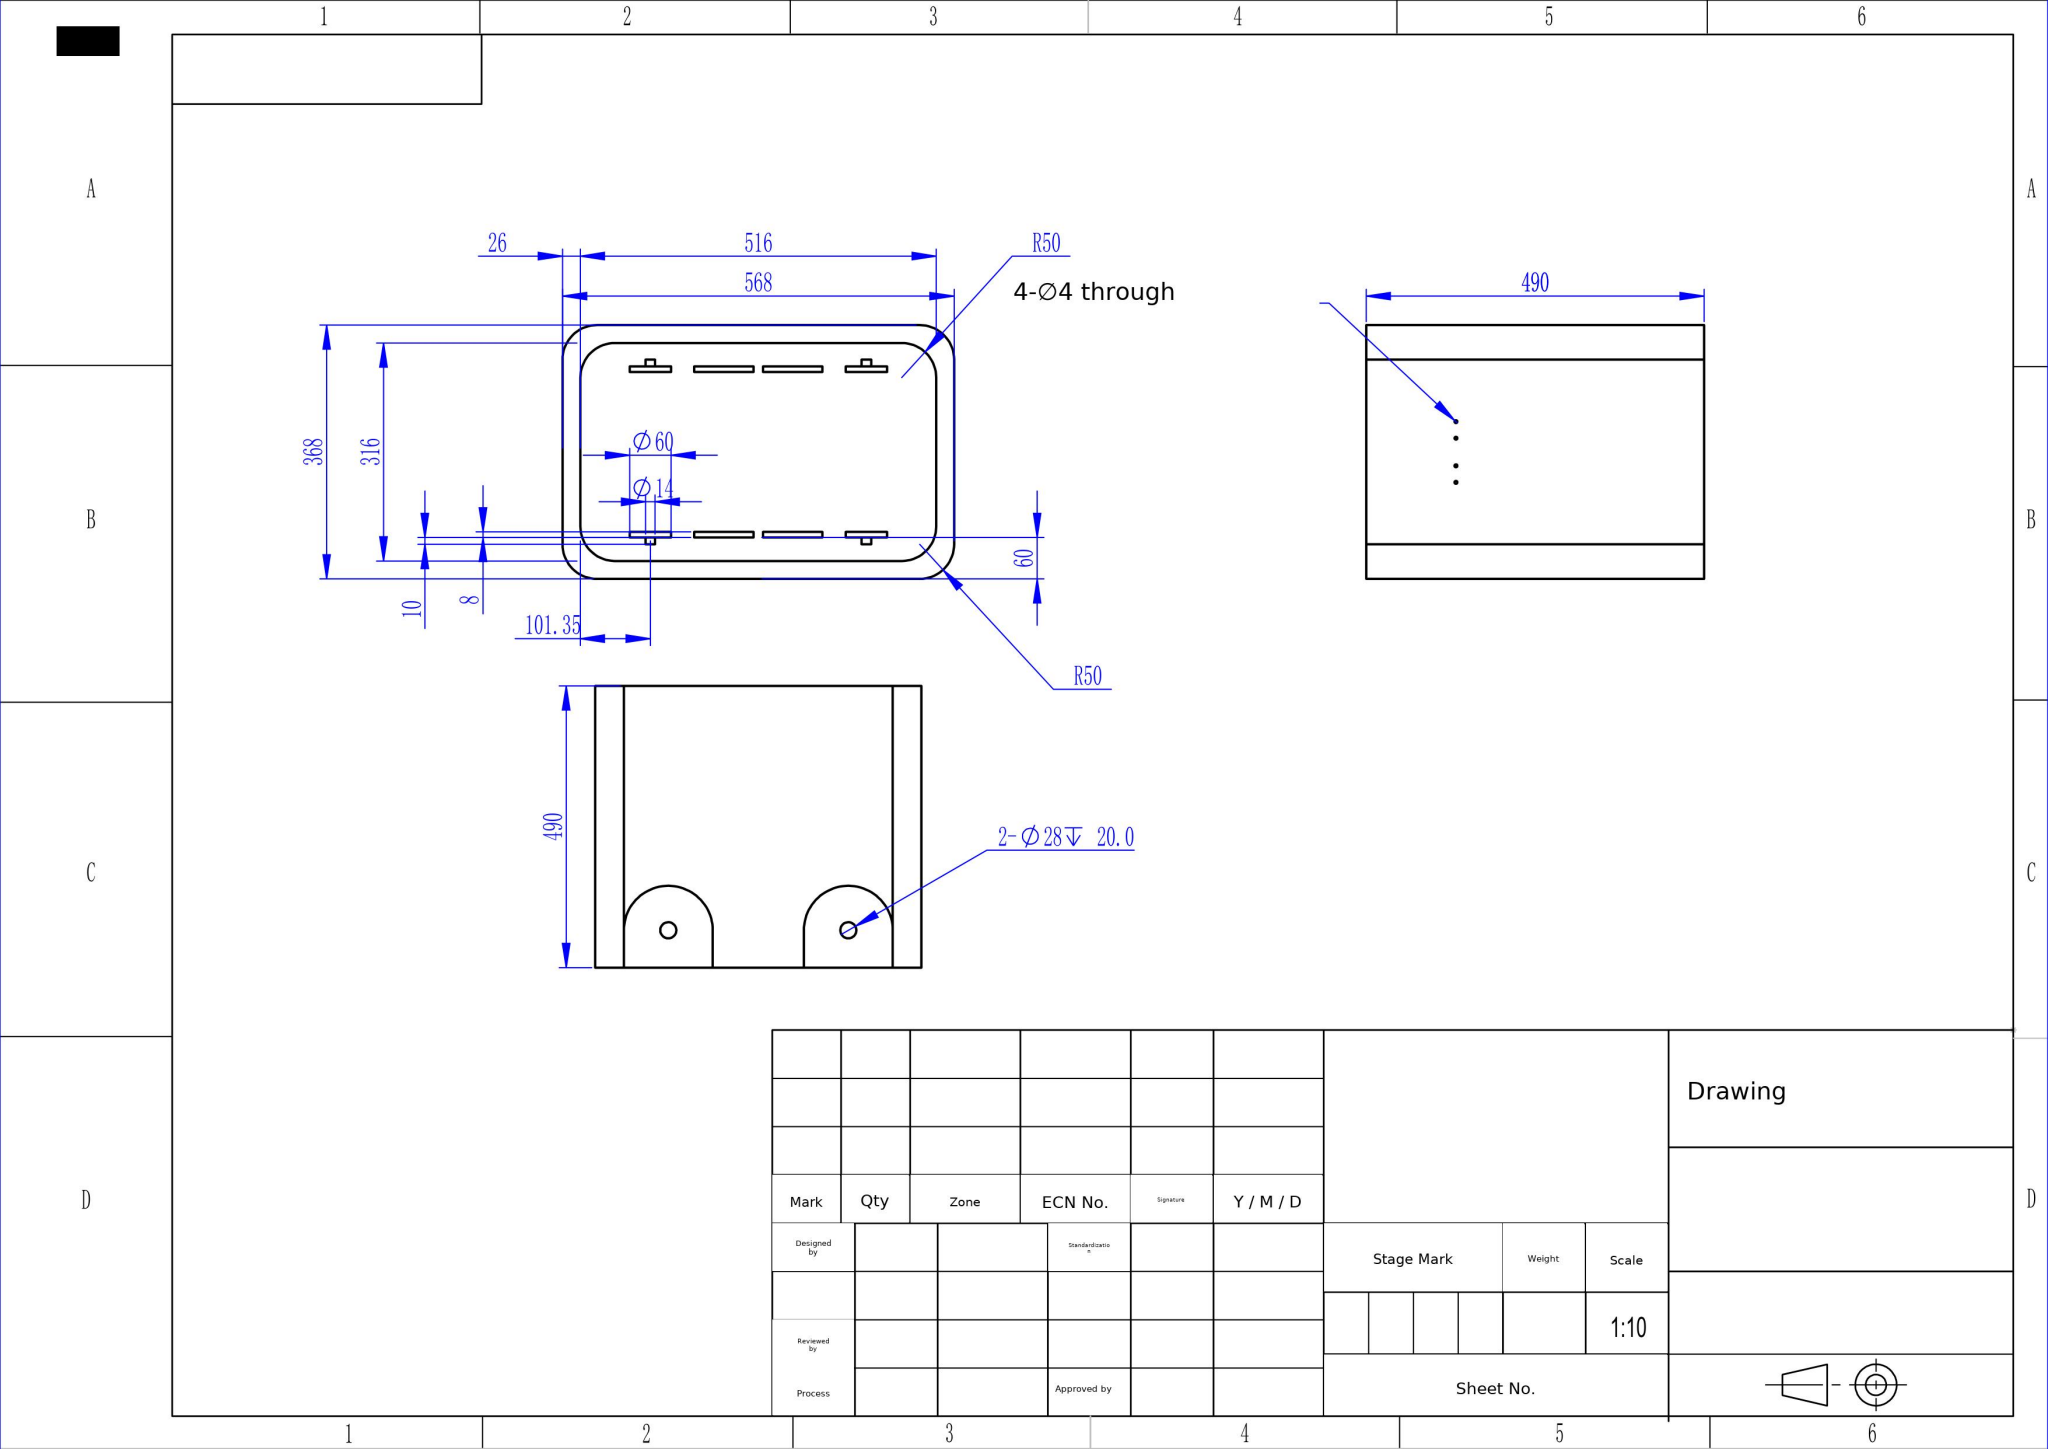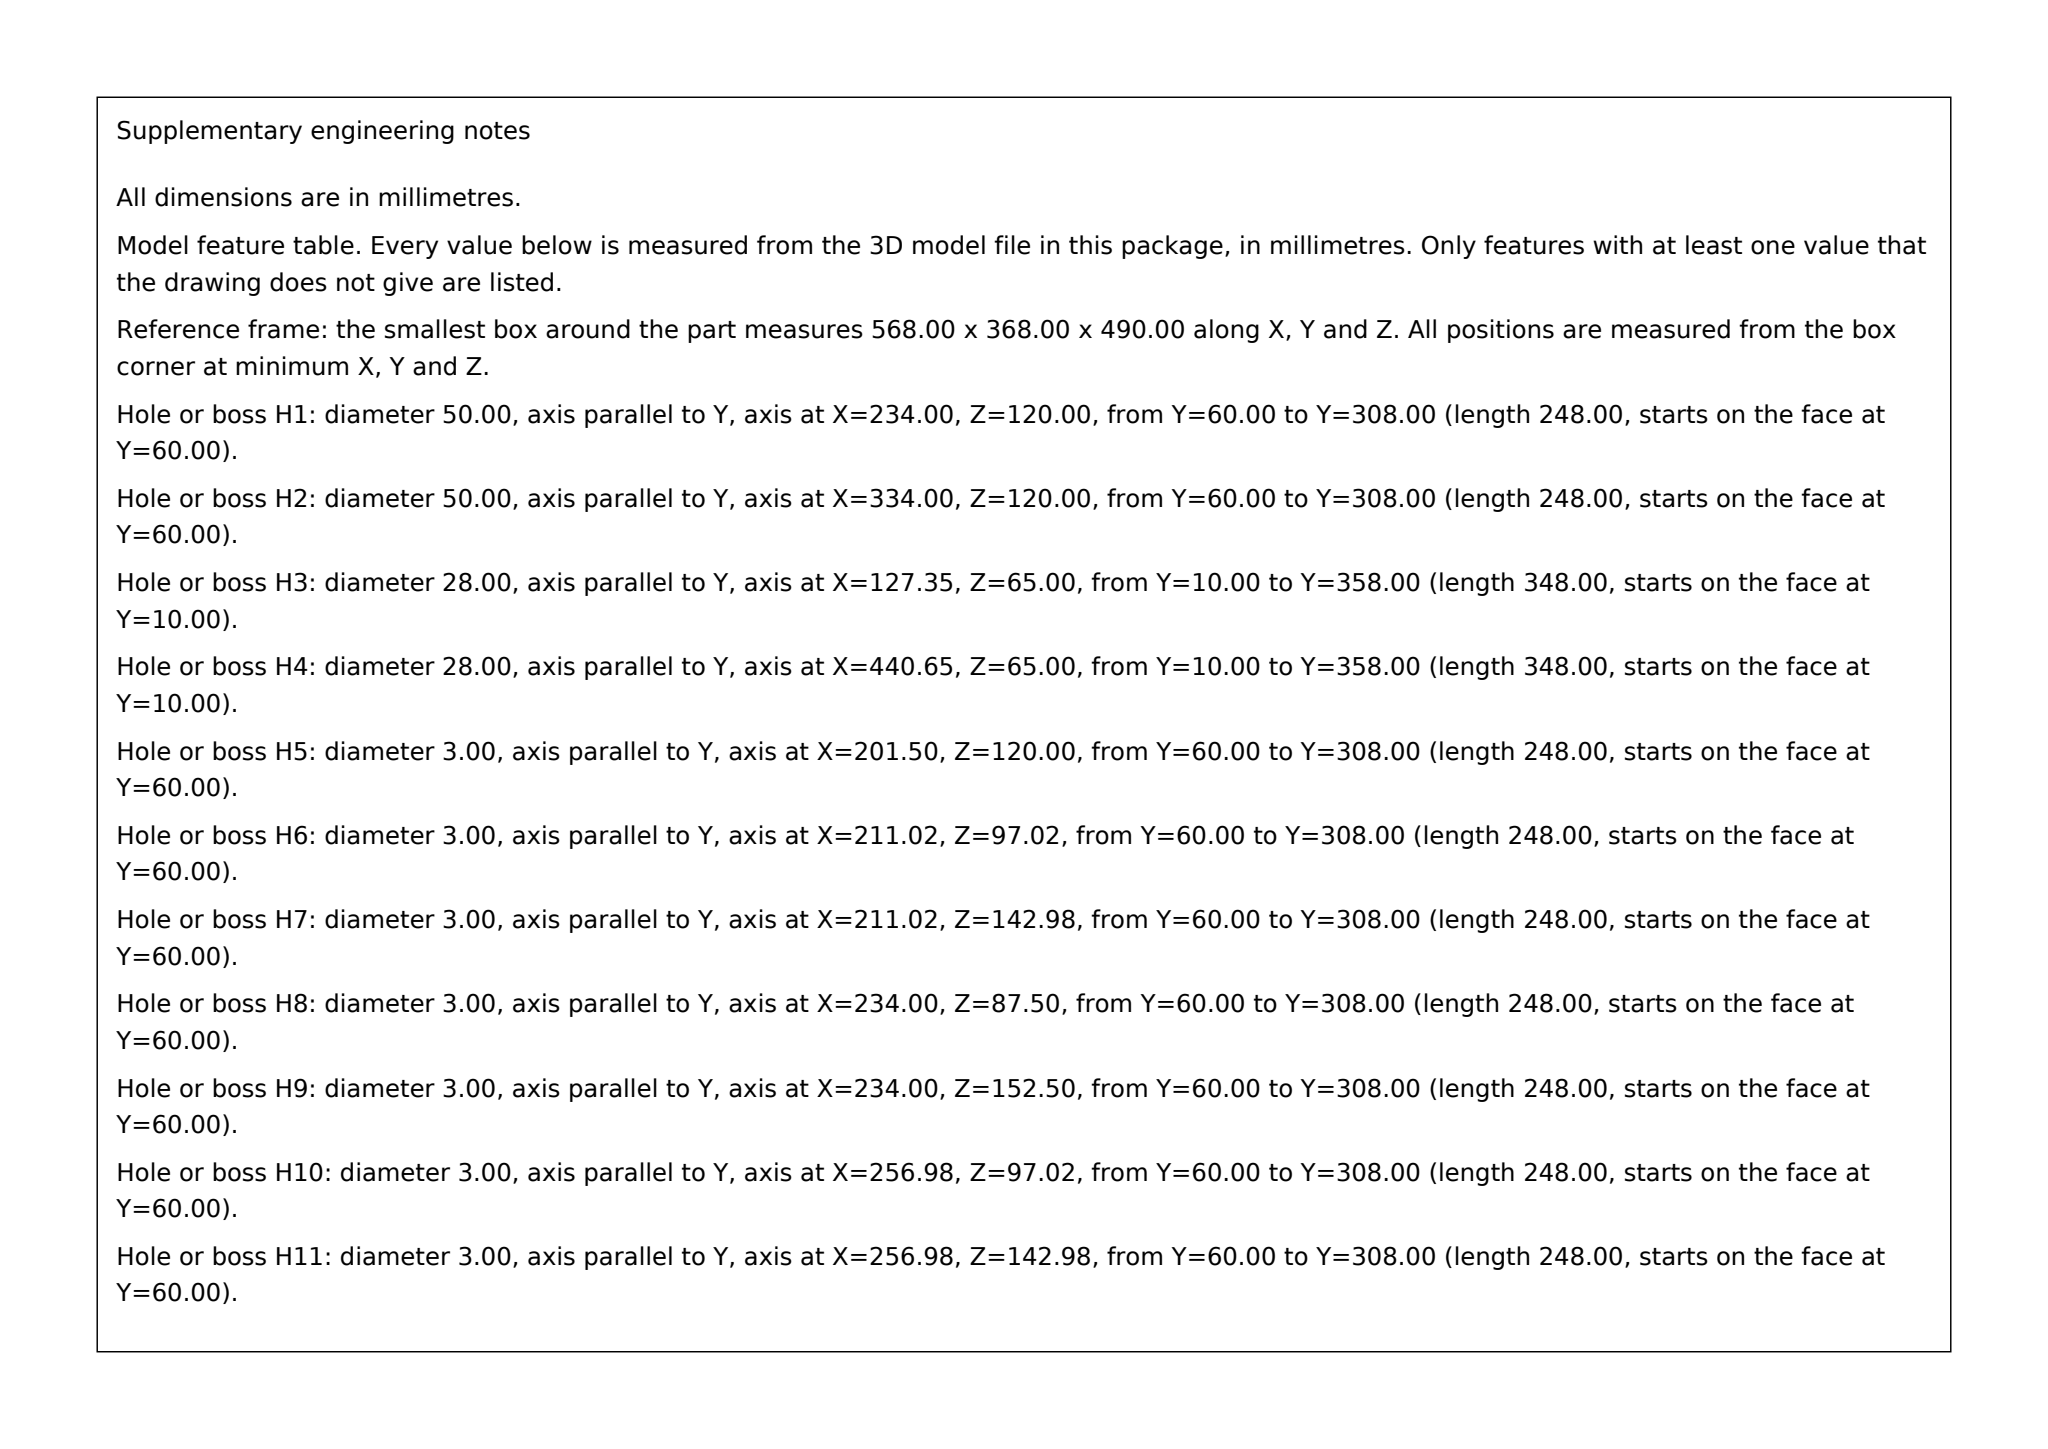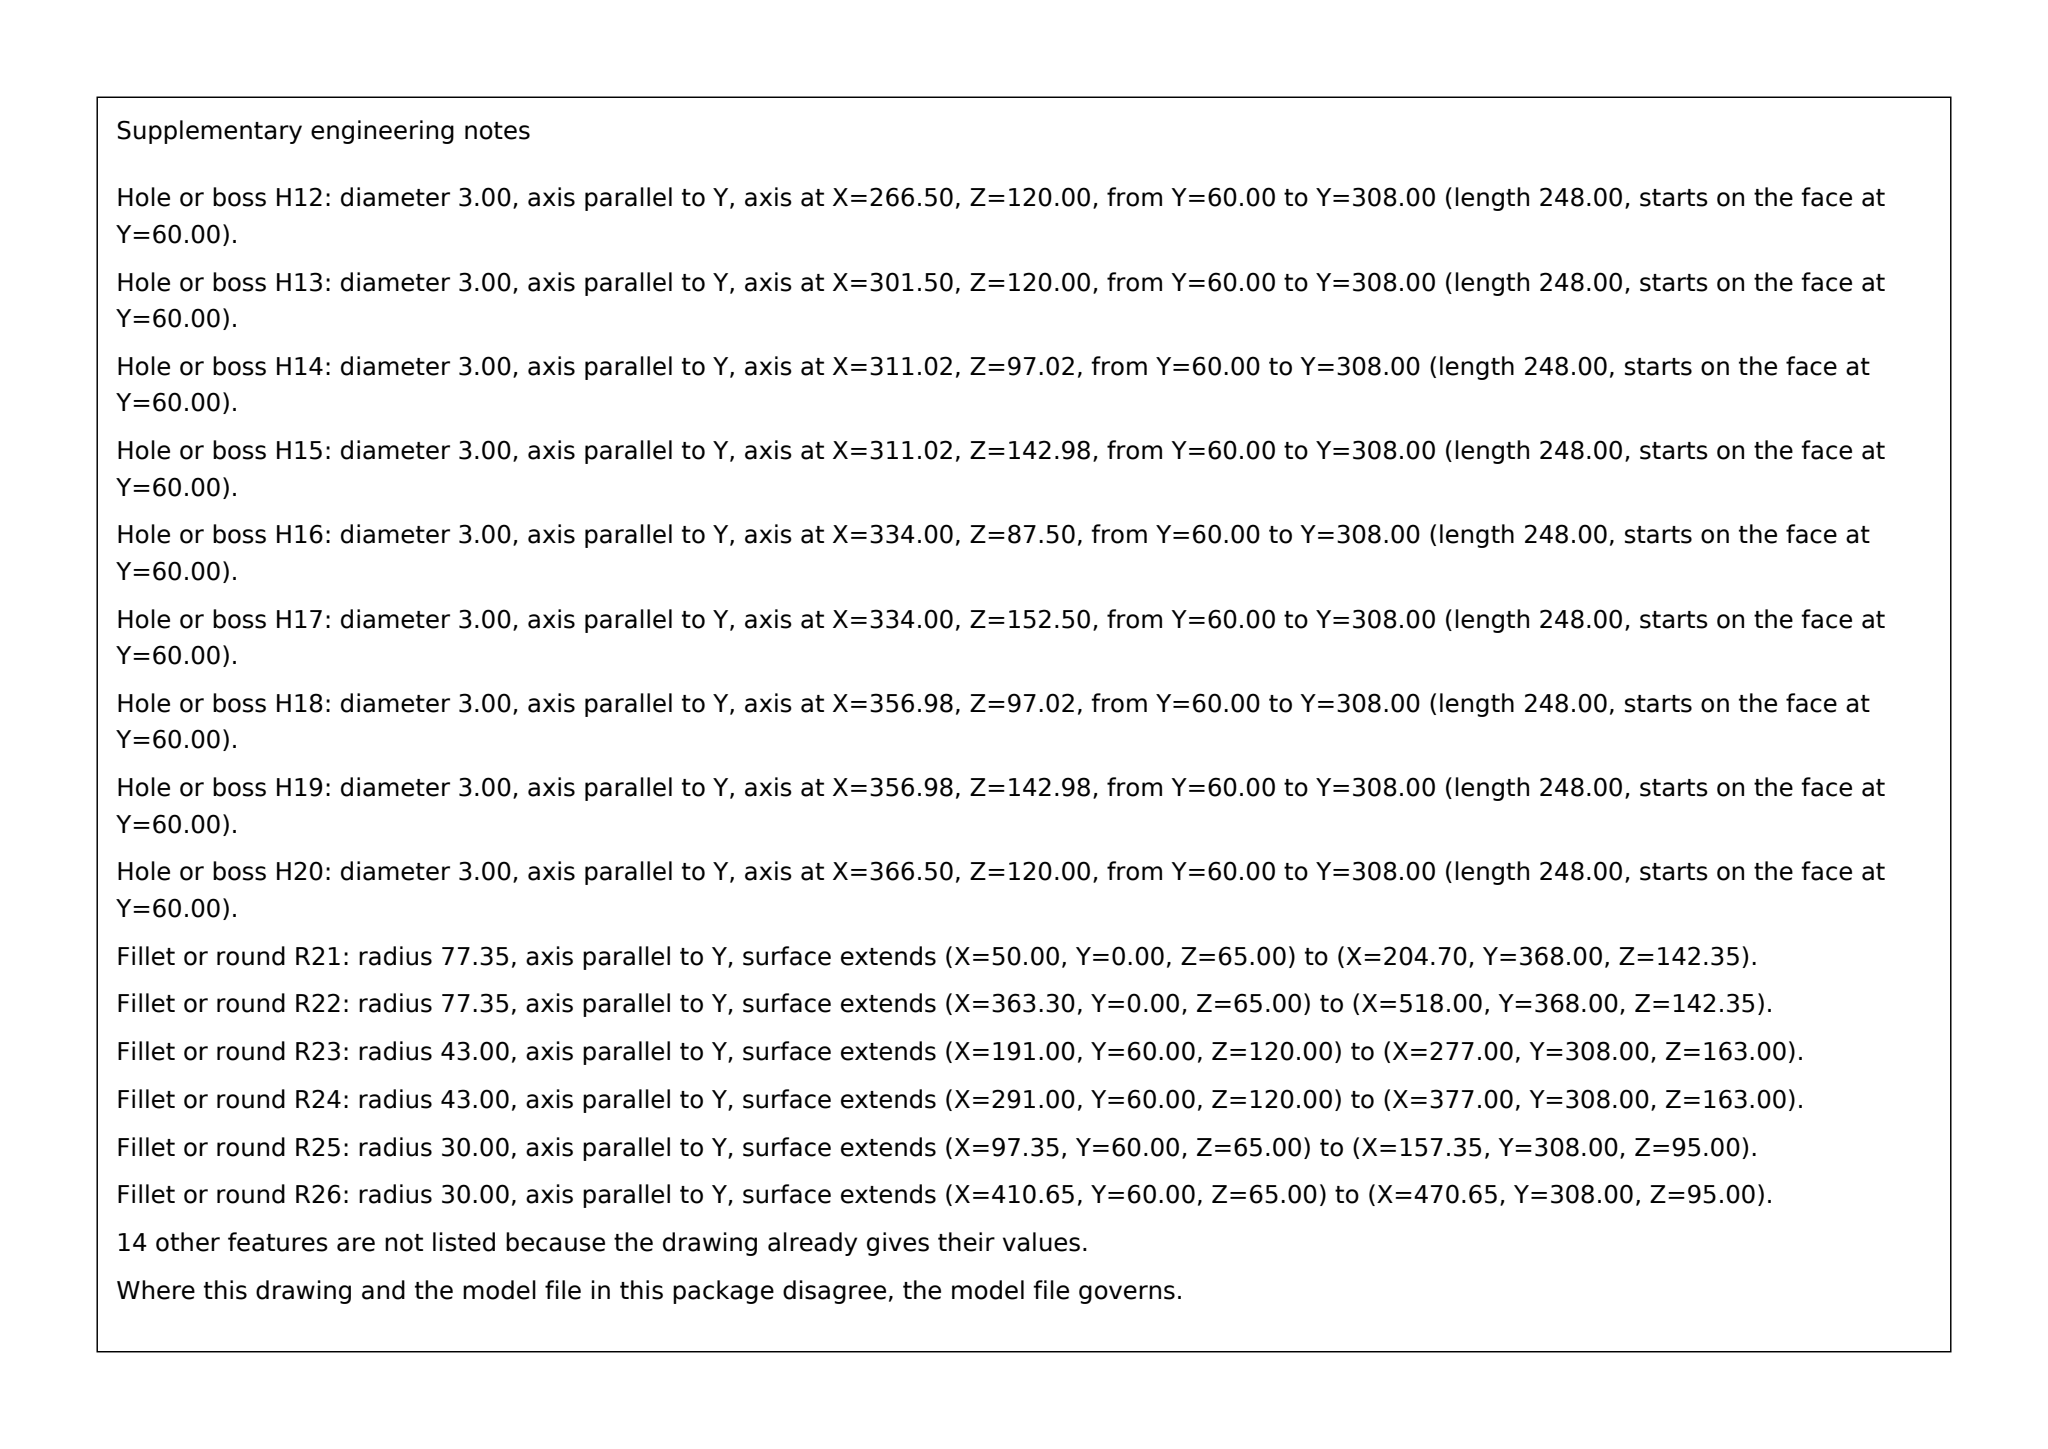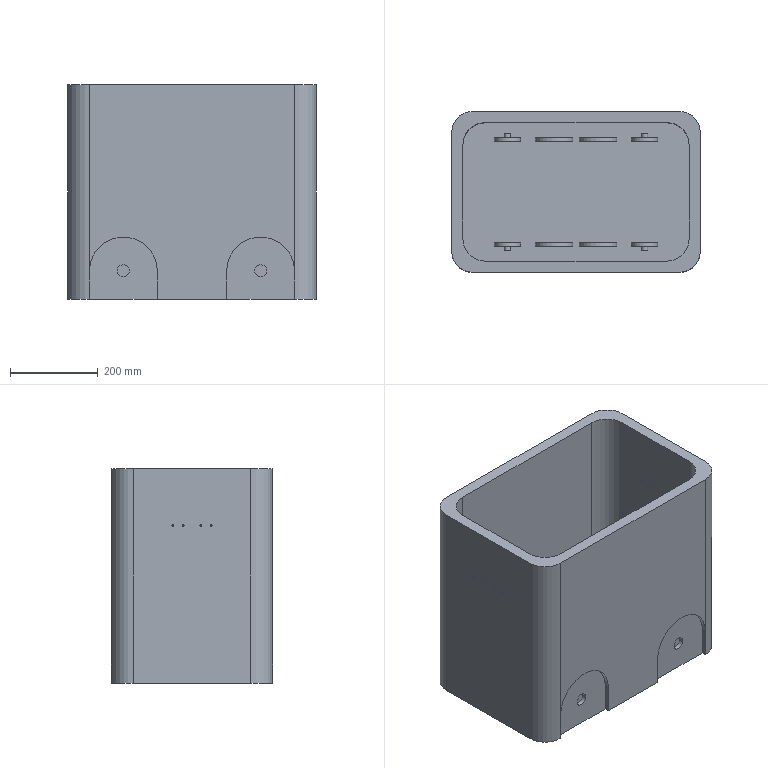Part | SolidWorks | mm | 1 solid | 187 faces | box 568 x 368 x 490 mm | volume 25378427 mm3 | cylinder 124 | plane 63 | commonest cylinder face diameters 3 x64 4 x16 28 x8 14 x8 50 x8 100 x8 86 x4 60 x4
build123d program:
from build123d import *

# Parameters (mm, degrees)
SKETCH2_W                 = 568
SKETCH2_H                 = 368
SKETCH2_W_2               = 516
SKETCH2_H_2               = 316
BOSS_EXTRUDE1_DEPTH       = 490
SKETCH3_W                 = 568
SKETCH3_H                 = 368
BOSS_EXTRUDE2_DEPTH       = 20
FILLET1_R                 = 50
FILLET2_R                 = 50
SKETCH6_R                 = 2
CUT_EXTRUDE6_DEPTH        = 773.386
SKETCH15_R                = 1.5
SKETCH15_R_2              = 25
BOSS_EXTRUDE3_DEPTH       = 8
BOSS_EXTRUDE4_DEPTH       = 8
SKETCH17_R                = 7
BOSS_EXTRUDE5_DEPTH       = 10
CUT_EXTRUDE11_START       = -10
SKETCH18_R                = 7
CUT_EXTRUDE11_DEPTH       = 10
SKETCH19_R                = 14
CUT_EXTRUDE12_DEPTH       = 20
MIRROR4_COPY_1_SKETCH_R   = 1.5
MIRROR4_COPY_1_SKETCH_R_2 = 25
MIRROR4_COPY_1_DEPTH      = 8
MIRROR4_COPY_2_DEPTH      = 8
MIRROR4_COPY_3_SKETCH_R   = 7
MIRROR4_COPY_3_DEPTH      = 10
MIRROR4_START             = -10
MIRROR4_COPY_4_SKETCH_R   = 7
MIRROR4_COPY_4_DEPTH      = 10
MIRROR4_COPY_5_SKETCH_R   = 14
MIRROR4_COPY_5_DEPTH      = 20


with BuildPart() as part:
    # Sketch2 → Boss-Extrude1 (new body)
    with BuildSketch(Plane.XY):
        Rectangle(SKETCH2_W, SKETCH2_H)
        Rectangle(SKETCH2_W_2, SKETCH2_H_2, mode=Mode.SUBTRACT)
    extrude(amount=BOSS_EXTRUDE1_DEPTH)

    # Sketch3 → Boss-Extrude2 (add)
    with BuildSketch(Plane(origin=(0, 0, 0), x_dir=(-1, 0, 0), z_dir=(0, 0, -1))):
        Rectangle(SKETCH3_W, SKETCH3_H)
    extrude(amount=-BOSS_EXTRUDE2_DEPTH)

    # Fillet1
    fillet1_edges = [part.edges().sort_by_distance(p)[0] for p in [
        (284, 184, 245),
        (284, -184, 245),
        (-284, -184, 245),
        (-284, 184, 245),
    ]]
    fillet(fillet1_edges, radius=FILLET1_R)

    # Fillet2
    fillet2_edges = [part.edges().sort_by_distance(p)[0] for p in [
        (258, -158, 255),
        (258, 158, 255),
        (-258, 158, 255),
        (-258, -158, 255),
    ]]
    fillet(fillet2_edges, radius=FILLET2_R)

    # Sketch6 → Cut-Extrude6 (cut, through all)
    with BuildSketch(Plane.ZY.offset(284)):
        with Locations((360, 44)):
            Circle(SKETCH6_R)
        with Locations((360, 20)):
            Circle(SKETCH6_R)
        with Locations(Location((360, -20, 0), (0, 0, 270))):
            Circle(SKETCH6_R)
        with Locations(Location((360, -44, 0), (0, 0, 270))):
            Circle(SKETCH6_R)
    extrude(amount=-CUT_EXTRUDE6_DEPTH, mode=Mode.SUBTRACT)

    # Sketch15 → Boss-Extrude3 (add)
    with BuildSketch(Plane(origin=(0, -124, 0), x_dir=(-1, 0, 0), z_dir=(0, -1, 0))):
        with BuildLine():
            Line((7, -20), (7, -120))
            ThreePointArc((7, -120), (50, -163), (93, -120))
            Line((93, -120), (93, -20))
            Line((93, -20), (7, -20))
        make_face()
        with Locations(Location((72.981, -97.019, 0), (0, 0, 180))):
            Circle(SKETCH15_R, mode=Mode.SUBTRACT)
        with Locations(Location((50, -87.5, 0), (0, 0, 180))):
            Circle(SKETCH15_R, mode=Mode.SUBTRACT)
        with Locations(Location((50, -120, 0), (0, 0, 180))):
            Circle(SKETCH15_R_2, mode=Mode.SUBTRACT)
        with Locations(Location((27.019, -97.019, 0), (0, 0, 180))):
            Circle(SKETCH15_R, mode=Mode.SUBTRACT)
        with Locations(Location((17.5, -120, 0), (0, 0, 180))):
            Circle(SKETCH15_R, mode=Mode.SUBTRACT)
        with Locations(Location((27.019, -142.981, 0), (0, 0, 180))):
            Circle(SKETCH15_R, mode=Mode.SUBTRACT)
        with Locations(Location((50, -152.5, 0), (0, 0, 180))):
            Circle(SKETCH15_R, mode=Mode.SUBTRACT)
        with Locations(Location((72.981, -142.981, 0), (0, 0, 180))):
            Circle(SKETCH15_R, mode=Mode.SUBTRACT)
        with Locations(Location((82.5, -120, 0), (0, 0, 180))):
            Circle(SKETCH15_R, mode=Mode.SUBTRACT)
    boss_extrude3 = extrude(amount=-BOSS_EXTRUDE3_DEPTH)

    # Sketch16 → Boss-Extrude4 (add)
    with BuildSketch(Plane(origin=(0, -124, 0), x_dir=(-1, 0, 0), z_dir=(0, -1, 0))):
        with BuildLine():
            Line((126.65, -65), (126.65, -20))
            Line((126.65, -20), (186.65, -20))
            Line((186.65, -20), (186.65, -65))
            ThreePointArc((186.65, -65), (156.65, -95), (126.65, -65))
        make_face()
    boss_extrude4 = extrude(amount=-BOSS_EXTRUDE4_DEPTH)

    # Sketch17 → Boss-Extrude5 (add)
    with BuildSketch(Plane.XZ.offset(124)):
        with Locations((-156.65, 65)):
            Circle(SKETCH17_R)
    boss_extrude5 = extrude(amount=BOSS_EXTRUDE5_DEPTH)

    # Sketch18 → Cut-Extrude11 (cut)
    # profile 1 of 2: a face of its own
    with BuildSketch(Plane.XZ.offset(184).offset(CUT_EXTRUDE11_START)):
        with BuildLine():
            ThreePointArc((-79.3, 65), (-156.65, 142.35), (-234, 65))
            Line((-234, 65), (-234, 0))
            Line((-234, 0), (-79.3, 0))
            Line((-79.3, 0), (-79.3, 65))
        make_face()
        with Locations((-156.65, 65)):
            Circle(SKETCH18_R, mode=Mode.SUBTRACT)
    # profile 2 of 2: a face of its own
    with BuildSketch(Plane.XZ.offset(184).offset(CUT_EXTRUDE11_START)):
        with Locations((-156.65, 65)):
            Circle(SKETCH18_R)
    cut_extrude11 = extrude(amount=CUT_EXTRUDE11_DEPTH, mode=Mode.SUBTRACT)

    # Sketch19 → Cut-Extrude12 (cut)
    with BuildSketch(Plane.XZ.offset(184)):
        with Locations((-156.65, 65)):
            Circle(SKETCH19_R)
    cut_extrude12 = extrude(amount=-CUT_EXTRUDE12_DEPTH, mode=Mode.SUBTRACT)

    # Mirror3: Boss-Extrude3, Boss-Extrude4, Boss-Extrude5, Cut-Extrude11, Cut-Extrude12 across plane
    add(boss_extrude3.mirror(Plane(origin=(0, 0, 0), x_dir=(0, 0, 1), z_dir=(1, 0, 0))))
    add(boss_extrude4.mirror(Plane(origin=(0, 0, 0), x_dir=(0, 0, 1), z_dir=(1, 0, 0))))
    add(boss_extrude5.mirror(Plane(origin=(0, 0, 0), x_dir=(0, 0, 1), z_dir=(1, 0, 0))))
    add(cut_extrude11.mirror(Plane(origin=(0, 0, 0), x_dir=(0, 0, 1), z_dir=(1, 0, 0))), mode=Mode.SUBTRACT)
    add(cut_extrude12.mirror(Plane(origin=(0, 0, 0), x_dir=(0, 0, 1), z_dir=(1, 0, 0))), mode=Mode.SUBTRACT)

    # Mirror4: Boss-Extrude3, Boss-Extrude4, Boss-Extrude5, Cut-Extrude11, Cut-Extrude12 across plane
    add(boss_extrude3.mirror(Plane.ZX))
    add(boss_extrude4.mirror(Plane.ZX))
    add(boss_extrude5.mirror(Plane.ZX))
    add(cut_extrude11.mirror(Plane.ZX), mode=Mode.SUBTRACT)
    add(cut_extrude12.mirror(Plane.ZX), mode=Mode.SUBTRACT)

    # Mirror4 copy 1 sketch → Mirror4 copy 1 (add)
    with BuildSketch(Plane(origin=(0, 124, 0), x_dir=(1, 0, 0), z_dir=(0, 1, 0))):
        with BuildLine():
            Line((7, -20), (7, -120))
            ThreePointArc((7, -120), (50, -163), (93, -120))
            Line((93, -120), (93, -20))
            Line((93, -20), (7, -20))
        make_face()
        with Locations(Location((72.981, -97.019, 0), (0, 0, 180))):
            Circle(MIRROR4_COPY_1_SKETCH_R, mode=Mode.SUBTRACT)
        with Locations(Location((50, -87.5, 0), (0, 0, 180))):
            Circle(MIRROR4_COPY_1_SKETCH_R, mode=Mode.SUBTRACT)
        with Locations(Location((50, -120, 0), (0, 0, 180))):
            Circle(MIRROR4_COPY_1_SKETCH_R_2, mode=Mode.SUBTRACT)
        with Locations(Location((27.019, -97.019, 0), (0, 0, 180))):
            Circle(MIRROR4_COPY_1_SKETCH_R, mode=Mode.SUBTRACT)
        with Locations(Location((17.5, -120, 0), (0, 0, 180))):
            Circle(MIRROR4_COPY_1_SKETCH_R, mode=Mode.SUBTRACT)
        with Locations(Location((27.019, -142.981, 0), (0, 0, 180))):
            Circle(MIRROR4_COPY_1_SKETCH_R, mode=Mode.SUBTRACT)
        with Locations(Location((50, -152.5, 0), (0, 0, 180))):
            Circle(MIRROR4_COPY_1_SKETCH_R, mode=Mode.SUBTRACT)
        with Locations(Location((72.981, -142.981, 0), (0, 0, 180))):
            Circle(MIRROR4_COPY_1_SKETCH_R, mode=Mode.SUBTRACT)
        with Locations(Location((82.5, -120, 0), (0, 0, 180))):
            Circle(MIRROR4_COPY_1_SKETCH_R, mode=Mode.SUBTRACT)
    extrude(amount=-MIRROR4_COPY_1_DEPTH)

    # Mirror4 copy 2 sketch → Mirror4 copy 2 (add)
    with BuildSketch(Plane(origin=(0, 124, 0), x_dir=(1, 0, 0), z_dir=(0, 1, 0))):
        with BuildLine():
            Line((126.65, -65), (126.65, -20))
            Line((126.65, -20), (186.65, -20))
            Line((186.65, -20), (186.65, -65))
            ThreePointArc((186.65, -65), (156.65, -95), (126.65, -65))
        make_face()
    extrude(amount=-MIRROR4_COPY_2_DEPTH)

    # Mirror4 copy 3 sketch → Mirror4 copy 3 (add)
    with BuildSketch(Plane(origin=(0, 124, 0), x_dir=(-1, 0, 0), z_dir=(0, 1, 0))):
        with Locations((-156.65, 65)):
            Circle(MIRROR4_COPY_3_SKETCH_R)
    extrude(amount=MIRROR4_COPY_3_DEPTH)

    # Mirror4 copy 4 sketch → Mirror4 copy 4 (cut)
    # profile 1 of 2: a face of its own
    with BuildSketch(Plane(origin=(0, 184, 0), x_dir=(-1, 0, 0), z_dir=(0, 1, 0)).offset(MIRROR4_START)):
        with BuildLine():
            ThreePointArc((-79.3, 65), (-156.65, 142.35), (-234, 65))
            Line((-234, 65), (-234, 0))
            Line((-234, 0), (-79.3, 0))
            Line((-79.3, 0), (-79.3, 65))
        make_face()
        with Locations((-156.65, 65)):
            Circle(MIRROR4_COPY_4_SKETCH_R, mode=Mode.SUBTRACT)
    # profile 2 of 2: a face of its own
    with BuildSketch(Plane(origin=(0, 184, 0), x_dir=(-1, 0, 0), z_dir=(0, 1, 0)).offset(MIRROR4_START)):
        with Locations((-156.65, 65)):
            Circle(MIRROR4_COPY_4_SKETCH_R)
    extrude(amount=MIRROR4_COPY_4_DEPTH, mode=Mode.SUBTRACT)

    # Mirror4 copy 5 sketch → Mirror4 copy 5 (cut)
    with BuildSketch(Plane(origin=(0, 184, 0), x_dir=(-1, 0, 0), z_dir=(0, 1, 0))):
        with Locations((-156.65, 65)):
            Circle(MIRROR4_COPY_5_SKETCH_R)
    extrude(amount=-MIRROR4_COPY_5_DEPTH, mode=Mode.SUBTRACT)


solid = part.part